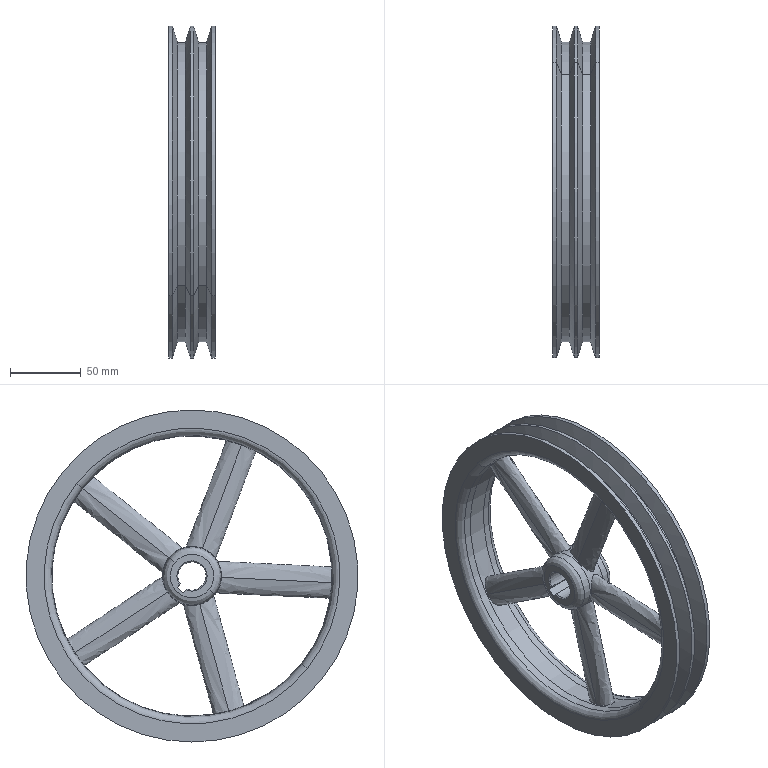Component | SolidWorks | V-beltLargeEllipticalSpokeWheel235x52.875x331-1 | 1 solid | 64 faces | volume 361035 mm3 | cone 22 | cylinder 17 | spline 10 | torus 8 | plane 7 | commonest cylinder face diameters 235 x6 212.1 x4 20 x3 41.732 x2 198.368 x2